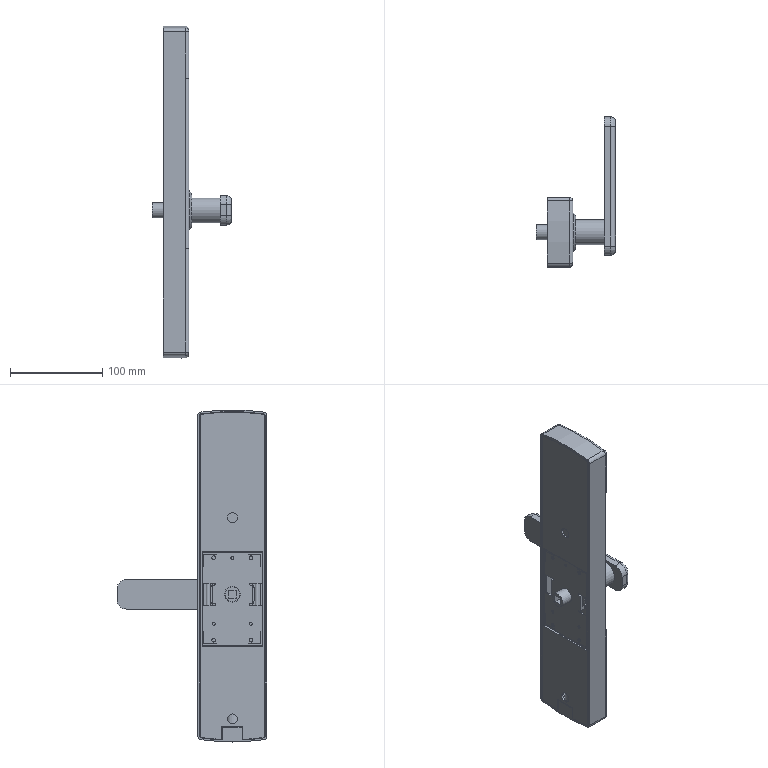Assembly | NX | mm | 16 component files | 16 solids | 730 faces | box 85.6 x 162.5 x 360 mm | volume 347839 mm3 | plane 400 | cylinder 166 | other 141 | torus 9 | sphere 8 | spline 4 | cone 2 | commonest cylinder face diameters 4 x32 8 x12 1.6 x12 2 x8 6 x8 5 x5 20 x5 2.2 x4
Bill of materials:
unnamed part 1 | 2 |  | Long, thin, plain solid cylindrical rod with flat ends.
unnamed part 2 | 1 |  | Square plate with rounded corners. One face carries a concentric circular feature with a stepped rim, which looks like a raised disc-shaped boss.
unnamed part 3 | 1 |  | Flat ring (washer-like) with a chamfered outer edge. The bore has two opposite rectangular notches and an internal step or counterbore.
unnamed part 4 | 1 |  | Long bar-shaped plate with fully rounded edges. A short stepped cylindrical stub sticks out at right angles from one face, near one end.
unnamed part 5 | 1 |  | Thin, long flat plate with gently arched short ends. It has a central rectangular window, two small round holes, and a rectangular notch in one end edge.
unnamed part 6 | 1 |  | Long bar-like body with arched ends and rounded edges. One face has a shallow recessed channel, two through holes (one of them in a small square raised pad), and narrow slots along the long edges.
unnamed part 7 | 1 |  | Flanged hub. A flat flange with chamfered corners and arched bulges top and bottom sits between a hollow stepped tubular shaft on one side and a larger stepped cylindrical boss with rectangular cut-outs on the other. A bore runs through.
unnamed part 8 | 1 |  | Straight link of uniform thickness: a thin web joining two round eyes, each with a through hole.
unnamed part 9 | 1 |  | Thin flat rectangular plate with sharp corners and one small round hole near each corner.
unnamed part 10 | 1 |  | Thin plate bracket with a stepped, notched outline. It has a large central round hole and several small holes. Two tabs are bent at right angles from the central part, each with a rectangular window and two small holes.
unnamed part 11 | 1 |  | Stepped cylindrical pin with a larger main body and a shorter, smaller end. The smaller end is split by a slot cut across it.
unnamed part 12 | 1 |  | Thick rectangular block with a large central through hole and four corner through holes. A shallow channel runs across one face.
unnamed part 13 | 1 |  | Cylindrical body with a smaller coaxial cylindrical boss on one end, a short reduced-diameter step on the other end, and two flat tabs on opposite sides. Each tab has rounded outer corners and one round through-hole.
unnamed part 14 | 1 |  | Plate of uniform thickness bent into a Z (joggle) shape. Two parallel end flanges are offset from each other and joined by a slanted middle section. The middle section has a large rectangular window, and each end flange has two round holes.
unnamed part 15 | 1 |  | Thin rectangular plate with rounded edges on the front. The front has shallow digit and symbol markings in a three-column grid. A single round through-hole near one end has an arc-shaped recess or chamfer around part of it. The back has a raised, slightly smaller rectangular pad.
Mates:
1. touch align | digital_panel 1 face | touch_housing 1 face
2. touch align | digital_panel 1 face | touch_housing 1 face
3. concentric | analog_fingerprint_button 1 edge | touch_housing 1 edge
4. concentric | spacer_block 1 edge | digital_panel 1 edge
5. touch align | housing 1 | touch_housing 1 face
6. distance | housing 1 face | spacer_block 1 face
7. center | slide_post 2 face | slide_post 2 face | housing 1 face | housing 1 face
8. distance | slide_post 2 face | housing 1 face
9. distance | slide_post 2 face | housing 1 face
10. bond | touch_housing 1 component | assembly component
11. bond | slide_post 2 component | assembly component
12. bond | slide_post 1 component | assembly component
13. linear | assembly datumaxis | assembly cartesiancoordinatesystem | assembly cartesiancoordinatesystem
14. touch align | push_plate 1 face | slide_post 2 face
15. touch align | push_plate 1 face | slide_post 1 face
16. fix | touch_housing 1 component
17. touch align | connecting_block 1 face | housing 1 face
18. distance | connecting_block 1 face | housing 1 face
19. concentric | selector_block 1 edge | connecting_block 1 edge
20. touch align | cover 1 face | housing 1 face
21. concentric | cover 1 edge | housing 1 edge
22. concentric | cover_plate 1 edge | touch_housing 1 edge
23. touch align | partition_plate 1 face | touch_housing 1 face
24. concentric | partition_plate 1 edge | touch_housing 1 edge
25. touch align | handle 1 face | connecting_block 1 face
26. distance | spacer_block 1 face | handle 1 face
27. concentric | safety_bolt 1 edge | touch_housing 1 edge
28. touch align | fixing_plate 1 face | touch_housing 1 face
29. touch align | fixing_plate 1 face | touch_housing 1 face
30. touch align | fixing_plate 1 face | touch_housing 1 face